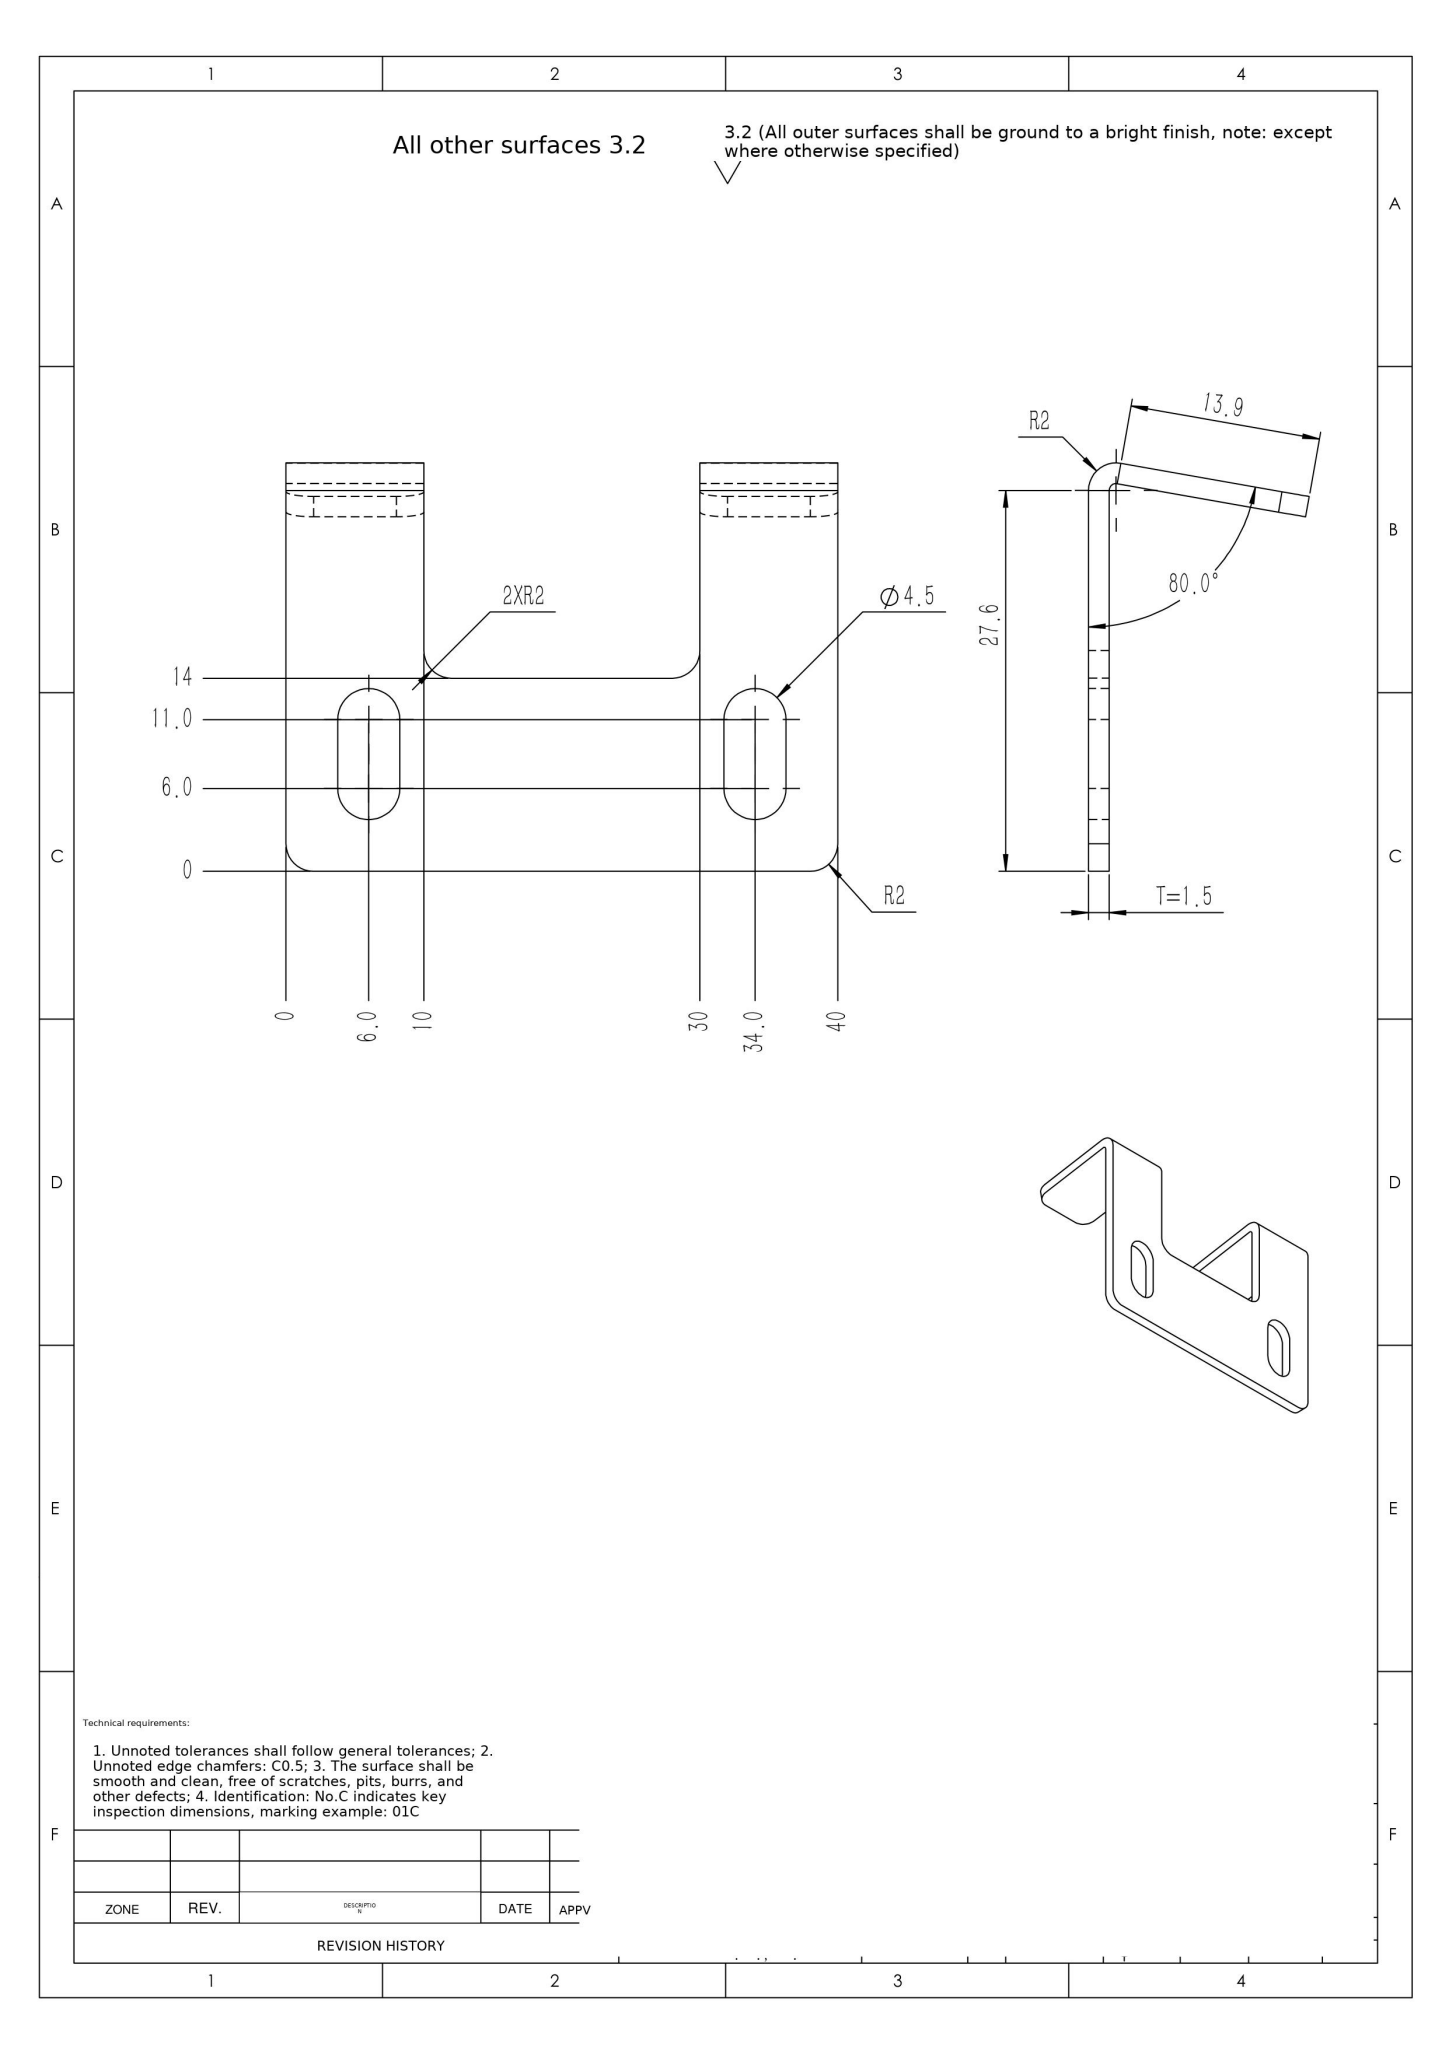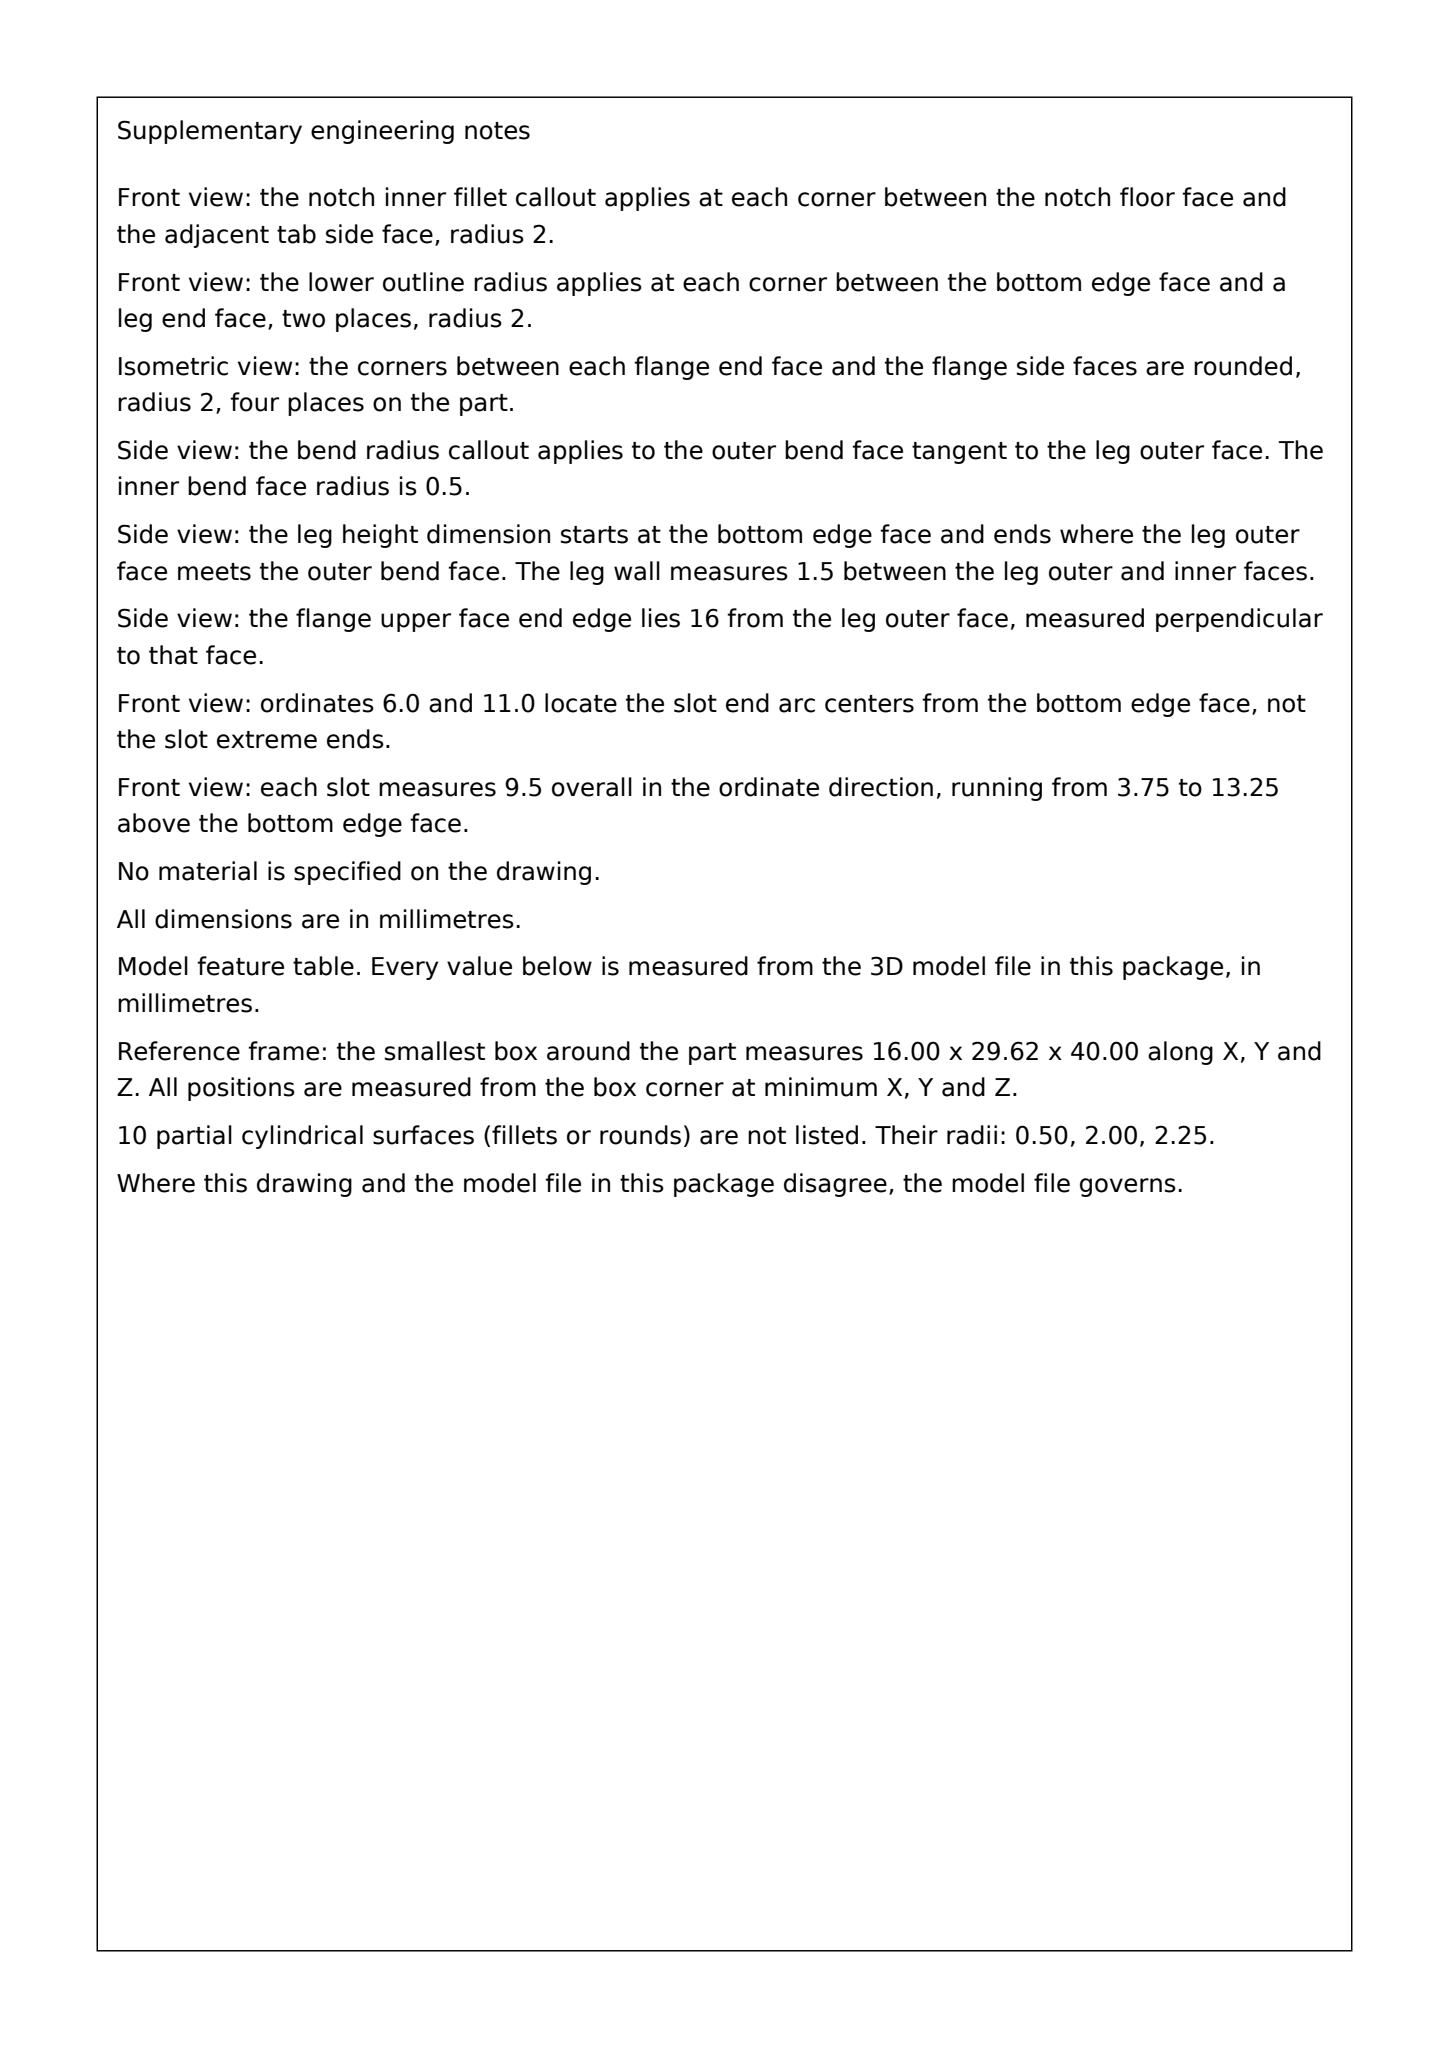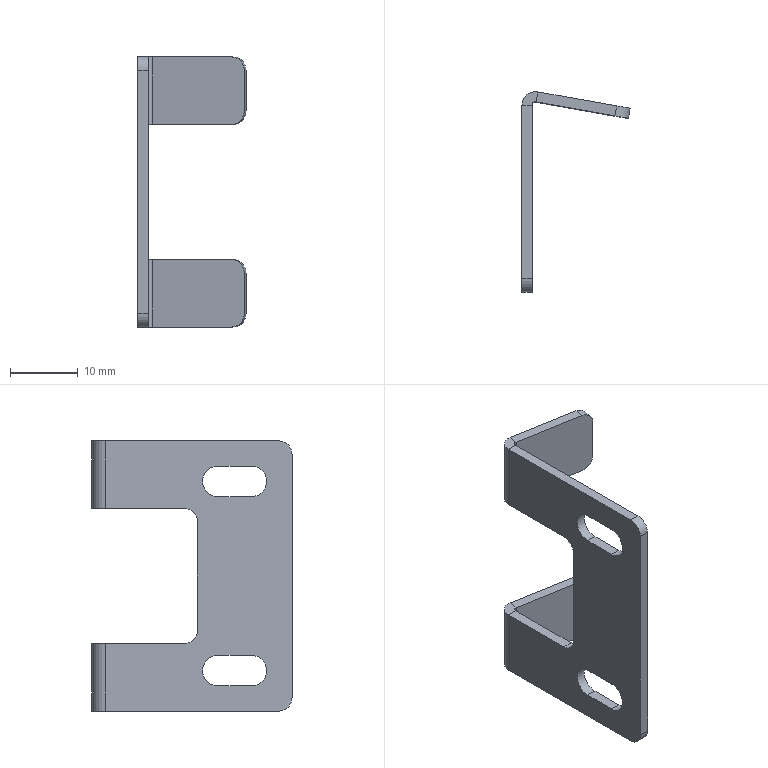Part | SolidWorks | mm | material Material | 1 solid | 44 faces | box 16 x 29.62 x 40 mm | volume 1609 mm3 | plane 26 | cylinder 18 | commonest cylinder face diameters 4 x10 4.5 x6 1 x2
Drawing notes:
FLANGE END OBLIQUE: CNRS 13.68 & 17.12 FROM PLATE BACK FACE | from the solid: 4X R2 y-axis cyl at x=13.68/z=2, x=17.12/z=8, x=14.03/z=38, x=17.12/z=32; plate faces x=0 & 1.5
OVERALL HT 29.6 FROM BTM EDGE (0) TO TOP OF BENT FLANGE | from the solid: bbox_xyz y=29.616; y-planes 0 & 14; bend R2 CL at y=27.62, x=2.0
TAB TIP 29.6 ABOVE BASE, 16.0 FROM BACK FACE | from the solid: bbox_xyz y=29.616 (=27.62+R2), x=16.0; base plane y=0, back face x=0
OVERALL DEPTH 16.0 FROM BACK FACE TO TAB TIP | from the solid: bbox_xyz x = 16.0, measured from x=0 back face plane
TAB ROOT AND BEND ZONE REMAIN FULL 10 WIDE (0-10 & 30-40 FROM LH EDGE): BEND R2 OUTSIDE / R0.5 INSIDE AXES AT 2.0 FROM BACK FACE, 27.62 ABOVE BTM EDGE, EACH 10.0 LONG | from the solid: cylinders [4.0, z, (2.0, 27.62), length 10, count 2] and [1.0, z, (2.0, 27.62), length 10, count 2]
4X R2 TAB TIP CORNERS: ROUND AXES VERTICAL AT 13.68 & 17.12 AND 14.03 & 17.12 FROM PLATE BACK FACE, AT 2.0/8.0 AND 32.0/38.0 FROM LH EDGE | from the solid: cylinders [4.0, y, (13.68, z=2.0)], [4.0, y, (14.03, z=38.0)], [4.0, y, (17.12, z=8.0)], [4.0, y, (17.12, z=32.0)], length 1.82
2X BENT TAB IS 10 WIDE FULL HEIGHT AND THROUGH BEND (Z 0-10 & 30-40 FROM LH EDGE); NO NARROWED SECTION ON TAB - 4.5 APPLIES TO SLOT WIDTH ONLY | from the solid: axis_planes z=0.0, 10.0, 30.0, 40.0 (3 each); bend cylinders dia 4.0 / dia 1.0 axis z at x=2.0, y=27.62, length 10.0 (2 each)